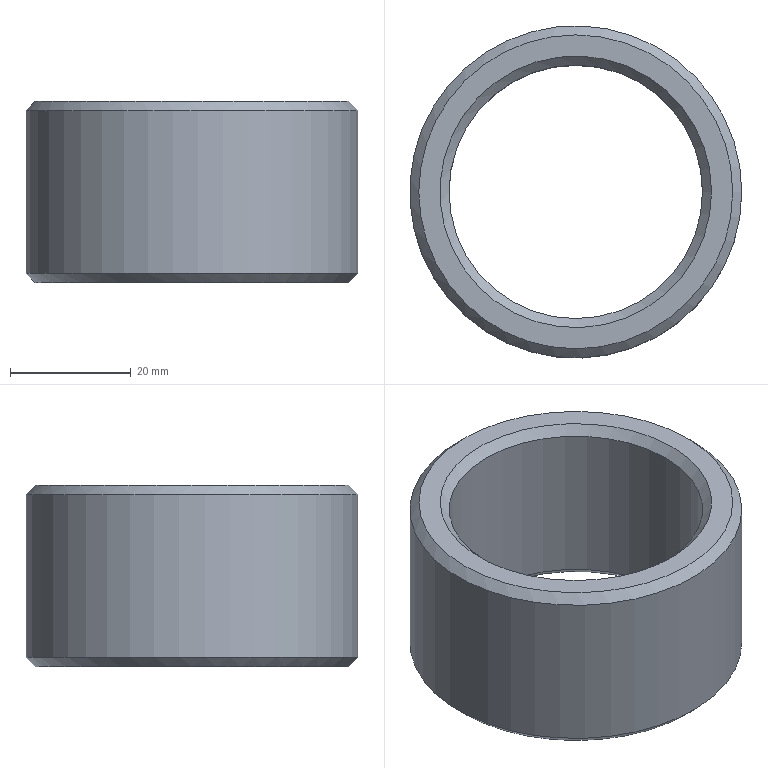Component | NX | BUSHING | 1 solid | 8 faces | box 55 x 55 x 30 mm | volume 29026 mm3 | cone 4 | cylinder 2 | plane 2 | commonest cylinder face diameters 55 x1 42 x1
STEP:
#1=CARTESIAN_POINT('',(0.,0.,0.));
#2=DIRECTION('',(0.,0.,1.));
#3=DIRECTION('',(1.,0.,0.));
#4=AXIS2_PLACEMENT_3D('',#1,#2,#3);
#5=CARTESIAN_POINT('',(61.5,144.033,51.5));
#6=VERTEX_POINT('',#5);
#7=CARTESIAN_POINT('',(34.,144.033,51.5));
#8=DIRECTION('',(0.,0.,1.));
#9=DIRECTION('',(1.,0.,0.));
#10=AXIS2_PLACEMENT_3D('',#7,#8,#9);
#11=CIRCLE('',#10,27.5);
#12=CARTESIAN_POINT('',(34.,144.033,80.));
#13=DIRECTION('',(0.,0.,-1.));
#14=DIRECTION('',(-1.,0.,0.));
#15=AXIS2_PLACEMENT_3D('',#12,#13,#14);
#16=CYLINDRICAL_SURFACE('',#15,27.5);
#17=CARTESIAN_POINT('',(9.425,28.5));
#18=DIRECTION('',(-1.,0.));
#19=VECTOR('',#18,1.);
#20=LINE('',#17,#19);
#21=(GEOMETRIC_REPRESENTATION_CONTEXT(2)PARAMETRIC_REPRESENTATION_CONTEXT()REPRESENTATION_CONTEXT('',''));
#22=DEFINITIONAL_REPRESENTATION('',(#20),#21);
#23=PCURVE('',#16,#22);
#24=CARTESIAN_POINT('',(34.,144.033,51.5));
#25=DIRECTION('',(0.,0.,1.));
#26=DIRECTION('',(1.,0.,0.));
#27=AXIS2_PLACEMENT_3D('',#24,#25,#26);
#28=CONICAL_SURFACE('',#27,27.5,0.7854);
#29=CARTESIAN_POINT('',(0.,0.));
#30=DIRECTION('',(1.,0.));
#31=VECTOR('',#30,1.);
#32=LINE('',#29,#31);
#33=(GEOMETRIC_REPRESENTATION_CONTEXT(2)PARAMETRIC_REPRESENTATION_CONTEXT()REPRESENTATION_CONTEXT('',''));
#34=DEFINITIONAL_REPRESENTATION('',(#32),#33);
#35=PCURVE('',#28,#34);
#36=SURFACE_CURVE('',#11,(#23,#35),.PCURVE_S1.);
#37=EDGE_CURVE('',#6,#6,#36,.T.);
#38=ORIENTED_EDGE('',*,*,#37,.T.);
#39=CARTESIAN_POINT('',(61.5,144.033,78.5));
#40=VERTEX_POINT('',#39);
#41=CARTESIAN_POINT('',(61.5,144.033,78.5));
#42=CARTESIAN_POINT('',(61.5,144.033,51.5));
#43=B_SPLINE_CURVE_WITH_KNOTS('',1,(#41,#42),.UNSPECIFIED.,.F.,.F.,(2,2),(1.5,28.5),.PIECEWISE_BEZIER_KNOTS.);
#44=CARTESIAN_POINT('',(3.142,0.));
#45=DIRECTION('',(0.,1.));
#46=VECTOR('',#45,1.);
#47=LINE('',#44,#46);
#48=(GEOMETRIC_REPRESENTATION_CONTEXT(2)PARAMETRIC_REPRESENTATION_CONTEXT()REPRESENTATION_CONTEXT('',''));
#49=DEFINITIONAL_REPRESENTATION('',(#47),#48);
#50=PCURVE('',#16,#49);
#51=CARTESIAN_POINT('',(9.425,0.));
#52=DIRECTION('',(0.,1.));
#53=VECTOR('',#52,1.);
#54=LINE('',#51,#53);
#55=(GEOMETRIC_REPRESENTATION_CONTEXT(2)PARAMETRIC_REPRESENTATION_CONTEXT()REPRESENTATION_CONTEXT('',''));
#56=DEFINITIONAL_REPRESENTATION('',(#54),#55);
#57=PCURVE('',#16,#56);
#58=SEAM_CURVE('',#43,(#50,#57),.PCURVE_S1.);
#59=EDGE_CURVE('',#40,#6,#58,.T.);
#60=ORIENTED_EDGE('',*,*,#59,.F.);
#61=CARTESIAN_POINT('',(34.,144.033,78.5));
#62=DIRECTION('',(0.,0.,-1.));
#63=DIRECTION('',(1.,0.,0.));
#64=AXIS2_PLACEMENT_3D('',#61,#62,#63);
#65=CIRCLE('',#64,27.5);
#66=CARTESIAN_POINT('',(3.142,1.5));
#67=DIRECTION('',(1.,0.));
#68=VECTOR('',#67,1.);
#69=LINE('',#66,#68);
#70=(GEOMETRIC_REPRESENTATION_CONTEXT(2)PARAMETRIC_REPRESENTATION_CONTEXT()REPRESENTATION_CONTEXT('',''));
#71=DEFINITIONAL_REPRESENTATION('',(#69),#70);
#72=PCURVE('',#16,#71);
#73=CARTESIAN_POINT('',(34.,144.033,80.));
#74=DIRECTION('',(0.,0.,-1.));
#75=DIRECTION('',(-1.,0.,0.));
#76=AXIS2_PLACEMENT_3D('',#73,#74,#75);
#77=CONICAL_SURFACE('',#76,26.,0.7854);
#78=CARTESIAN_POINT('',(3.142,1.5));
#79=DIRECTION('',(1.,0.));
#80=VECTOR('',#79,1.);
#81=LINE('',#78,#80);
#82=(GEOMETRIC_REPRESENTATION_CONTEXT(2)PARAMETRIC_REPRESENTATION_CONTEXT()REPRESENTATION_CONTEXT('',''));
#83=DEFINITIONAL_REPRESENTATION('',(#81),#82);
#84=PCURVE('',#77,#83);
#85=SURFACE_CURVE('',#65,(#72,#84),.PCURVE_S1.);
#86=EDGE_CURVE('',#40,#40,#85,.T.);
#87=ORIENTED_EDGE('',*,*,#86,.T.);
#88=ORIENTED_EDGE('',*,*,#59,.T.);
#89=EDGE_LOOP('',(#38,#60,#87,#88));
#90=FACE_BOUND('',#89,.T.);
#91=ADVANCED_FACE('',(#90),#16,.T.);
#92=CARTESIAN_POINT('',(55.,144.033,51.5));
#93=VERTEX_POINT('',#92);
#94=CARTESIAN_POINT('',(34.,144.033,51.5));
#95=DIRECTION('',(0.,0.,-1.));
#96=DIRECTION('',(1.,0.,0.));
#97=AXIS2_PLACEMENT_3D('',#94,#95,#96);
#98=CIRCLE('',#97,21.);
#99=CARTESIAN_POINT('',(34.,144.033,80.));
#100=DIRECTION('',(0.,0.,-1.));
#101=DIRECTION('',(-1.,0.,0.));
#102=AXIS2_PLACEMENT_3D('',#99,#100,#101);
#103=CYLINDRICAL_SURFACE('',#102,21.);
#104=CARTESIAN_POINT('',(3.142,28.5));
#105=DIRECTION('',(1.,0.));
#106=VECTOR('',#105,1.);
#107=LINE('',#104,#106);
#108=(GEOMETRIC_REPRESENTATION_CONTEXT(2)PARAMETRIC_REPRESENTATION_CONTEXT()REPRESENTATION_CONTEXT('',''));
#109=DEFINITIONAL_REPRESENTATION('',(#107),#108);
#110=PCURVE('',#103,#109);
#111=CARTESIAN_POINT('',(34.,144.033,50.));
#112=DIRECTION('',(0.,0.,-1.));
#113=DIRECTION('',(-1.,0.,0.));
#114=AXIS2_PLACEMENT_3D('',#111,#112,#113);
#115=CONICAL_SURFACE('',#114,22.5,0.7854);
#116=CARTESIAN_POINT('',(3.142,-1.5));
#117=DIRECTION('',(1.,0.));
#118=VECTOR('',#117,1.);
#119=LINE('',#116,#118);
#120=(GEOMETRIC_REPRESENTATION_CONTEXT(2)PARAMETRIC_REPRESENTATION_CONTEXT()REPRESENTATION_CONTEXT('',''));
#121=DEFINITIONAL_REPRESENTATION('',(#119),#120);
#122=PCURVE('',#115,#121);
#123=SURFACE_CURVE('',#98,(#110,#122),.PCURVE_S1.);
#124=EDGE_CURVE('',#93,#93,#123,.T.);
#125=ORIENTED_EDGE('',*,*,#124,.F.);
#126=CARTESIAN_POINT('',(55.,144.033,78.5));
#127=VERTEX_POINT('',#126);
#128=CARTESIAN_POINT('',(55.,144.033,78.5));
#129=CARTESIAN_POINT('',(55.,144.033,51.5));
#130=B_SPLINE_CURVE_WITH_KNOTS('',1,(#128,#129),.UNSPECIFIED.,.F.,.F.,(2,2),(1.5,28.5),.PIECEWISE_BEZIER_KNOTS.);
#131=CARTESIAN_POINT('',(3.142,0.));
#132=DIRECTION('',(0.,1.));
#133=VECTOR('',#132,1.);
#134=LINE('',#131,#133);
#135=(GEOMETRIC_REPRESENTATION_CONTEXT(2)PARAMETRIC_REPRESENTATION_CONTEXT()REPRESENTATION_CONTEXT('',''));
#136=DEFINITIONAL_REPRESENTATION('',(#134),#135);
#137=PCURVE('',#103,#136);
#138=CARTESIAN_POINT('',(9.425,0.));
#139=DIRECTION('',(0.,1.));
#140=VECTOR('',#139,1.);
#141=LINE('',#138,#140);
#142=(GEOMETRIC_REPRESENTATION_CONTEXT(2)PARAMETRIC_REPRESENTATION_CONTEXT()REPRESENTATION_CONTEXT('',''));
#143=DEFINITIONAL_REPRESENTATION('',(#141),#142);
#144=PCURVE('',#103,#143);
#145=SEAM_CURVE('',#130,(#137,#144),.PCURVE_S1.);
#146=EDGE_CURVE('',#127,#93,#145,.T.);
#147=ORIENTED_EDGE('',*,*,#146,.F.);
#148=CARTESIAN_POINT('',(34.,144.033,78.5));
#149=DIRECTION('',(0.,0.,1.));
#150=DIRECTION('',(1.,0.,0.));
#151=AXIS2_PLACEMENT_3D('',#148,#149,#150);
#152=CIRCLE('',#151,21.);
#153=CARTESIAN_POINT('',(9.425,1.5));
#154=DIRECTION('',(-1.,0.));
#155=VECTOR('',#154,1.);
#156=LINE('',#153,#155);
#157=(GEOMETRIC_REPRESENTATION_CONTEXT(2)PARAMETRIC_REPRESENTATION_CONTEXT()REPRESENTATION_CONTEXT('',''));
#158=DEFINITIONAL_REPRESENTATION('',(#156),#157);
#159=PCURVE('',#103,#158);
#160=CARTESIAN_POINT('',(34.,144.033,78.5));
#161=DIRECTION('',(0.,0.,1.));
#162=DIRECTION('',(1.,0.,0.));
#163=AXIS2_PLACEMENT_3D('',#160,#161,#162);
#164=CONICAL_SURFACE('',#163,21.,0.7854);
#165=CARTESIAN_POINT('',(0.,0.));
#166=DIRECTION('',(1.,0.));
#167=VECTOR('',#166,1.);
#168=LINE('',#165,#167);
#169=(GEOMETRIC_REPRESENTATION_CONTEXT(2)PARAMETRIC_REPRESENTATION_CONTEXT()REPRESENTATION_CONTEXT('',''));
#170=DEFINITIONAL_REPRESENTATION('',(#168),#169);
#171=PCURVE('',#164,#170);
#172=SURFACE_CURVE('',#152,(#159,#171),.PCURVE_S1.);
#173=EDGE_CURVE('',#127,#127,#172,.T.);
#174=ORIENTED_EDGE('',*,*,#173,.F.);
#175=ORIENTED_EDGE('',*,*,#146,.T.);
#176=EDGE_LOOP('',(#125,#147,#174,#175));
#177=FACE_BOUND('',#176,.F.);
#178=ADVANCED_FACE('',(#177),#103,.F.);
#179=CARTESIAN_POINT('',(56.5,144.033,80.));
#180=VERTEX_POINT('',#179);
#181=CARTESIAN_POINT('',(34.,144.033,80.));
#182=DIRECTION('',(0.,0.,-1.));
#183=DIRECTION('',(1.,0.,0.));
#184=AXIS2_PLACEMENT_3D('',#181,#182,#183);
#185=CIRCLE('',#184,22.5);
#186=CARTESIAN_POINT('',(34.,144.033,80.));
#187=DIRECTION('',(0.,0.,1.));
#188=DIRECTION('',(1.,0.,0.));
#189=AXIS2_PLACEMENT_3D('',#186,#187,#188);
#190=PLANE('',#189);
#191=CARTESIAN_POINT('',(22.5,0.));
#192=CARTESIAN_POINT('',(22.5,-38.971));
#193=CARTESIAN_POINT('',(-11.25,-19.486));
#194=CARTESIAN_POINT('',(-45.,-0.));
#195=CARTESIAN_POINT('',(-11.25,19.486));
#196=CARTESIAN_POINT('',(22.5,38.971));
#197=CARTESIAN_POINT('',(22.5,0.));
#198=(BOUNDED_CURVE()B_SPLINE_CURVE(2,(#191,#192,#193,#194,#195,#196,#197),.UNSPECIFIED.,.T.,.F.)B_SPLINE_CURVE_WITH_KNOTS((1,2,2,2,2,1),(-2.094,0.,2.094,4.189,6.283,8.378),.UNSPECIFIED.)CURVE()GEOMETRIC_REPRESENTATION_ITEM()RATIONAL_B_SPLINE_CURVE((1.,0.5,1.,0.5,1.,0.5,1.))REPRESENTATION_ITEM(''));
#199=(GEOMETRIC_REPRESENTATION_CONTEXT(2)PARAMETRIC_REPRESENTATION_CONTEXT()REPRESENTATION_CONTEXT('',''));
#200=DEFINITIONAL_REPRESENTATION('',(#198),#199);
#201=PCURVE('',#190,#200);
#202=CARTESIAN_POINT('',(6.283,1.5));
#203=DIRECTION('',(-1.,0.));
#204=VECTOR('',#203,1.);
#205=LINE('',#202,#204);
#206=(GEOMETRIC_REPRESENTATION_CONTEXT(2)PARAMETRIC_REPRESENTATION_CONTEXT()REPRESENTATION_CONTEXT('',''));
#207=DEFINITIONAL_REPRESENTATION('',(#205),#206);
#208=PCURVE('',#164,#207);
#209=SURFACE_CURVE('',#185,(#201,#208),.PCURVE_S1.);
#210=EDGE_CURVE('',#180,#180,#209,.T.);
#211=ORIENTED_EDGE('',*,*,#210,.T.);
#212=EDGE_LOOP('',(#211));
#213=FACE_BOUND('',#212,.T.);
#214=CARTESIAN_POINT('',(60.,144.033,80.));
#215=VERTEX_POINT('',#214);
#216=CARTESIAN_POINT('',(34.,144.033,80.));
#217=DIRECTION('',(0.,0.,1.));
#218=DIRECTION('',(1.,0.,0.));
#219=AXIS2_PLACEMENT_3D('',#216,#217,#218);
#220=CIRCLE('',#219,26.);
#221=CARTESIAN_POINT('',(0.,0.));
#222=DIRECTION('',(1.,0.));
#223=AXIS2_PLACEMENT_2D('',#221,#222);
#224=CIRCLE('',#223,26.);
#225=(GEOMETRIC_REPRESENTATION_CONTEXT(2)PARAMETRIC_REPRESENTATION_CONTEXT()REPRESENTATION_CONTEXT('',''));
#226=DEFINITIONAL_REPRESENTATION('',(#224),#225);
#227=PCURVE('',#190,#226);
#228=CARTESIAN_POINT('',(9.425,0.));
#229=DIRECTION('',(-1.,0.));
#230=VECTOR('',#229,1.);
#231=LINE('',#228,#230);
#232=(GEOMETRIC_REPRESENTATION_CONTEXT(2)PARAMETRIC_REPRESENTATION_CONTEXT()REPRESENTATION_CONTEXT('',''));
#233=DEFINITIONAL_REPRESENTATION('',(#231),#232);
#234=PCURVE('',#77,#233);
#235=SURFACE_CURVE('',#220,(#227,#234),.PCURVE_S1.);
#236=EDGE_CURVE('',#215,#215,#235,.T.);
#237=ORIENTED_EDGE('',*,*,#236,.T.);
#238=EDGE_LOOP('',(#237));
#239=FACE_BOUND('',#238,.T.);
#240=ADVANCED_FACE('',(#213,#239),#190,.T.);
#241=CARTESIAN_POINT('',(56.5,144.033,50.));
#242=VERTEX_POINT('',#241);
#243=CARTESIAN_POINT('',(34.,144.033,50.));
#244=DIRECTION('',(0.,0.,1.));
#245=DIRECTION('',(1.,0.,0.));
#246=AXIS2_PLACEMENT_3D('',#243,#244,#245);
#247=CIRCLE('',#246,22.5);
#248=CARTESIAN_POINT('',(34.,144.033,50.));
#249=DIRECTION('',(0.,0.,1.));
#250=DIRECTION('',(1.,0.,0.));
#251=AXIS2_PLACEMENT_3D('',#248,#249,#250);
#252=PLANE('',#251);
#253=CARTESIAN_POINT('',(0.,0.));
#254=DIRECTION('',(1.,0.));
#255=AXIS2_PLACEMENT_2D('',#253,#254);
#256=CIRCLE('',#255,22.5);
#257=(GEOMETRIC_REPRESENTATION_CONTEXT(2)PARAMETRIC_REPRESENTATION_CONTEXT()REPRESENTATION_CONTEXT('',''));
#258=DEFINITIONAL_REPRESENTATION('',(#256),#257);
#259=PCURVE('',#252,#258);
#260=CARTESIAN_POINT('',(9.425,0.));
#261=DIRECTION('',(-1.,0.));
#262=VECTOR('',#261,1.);
#263=LINE('',#260,#262);
#264=(GEOMETRIC_REPRESENTATION_CONTEXT(2)PARAMETRIC_REPRESENTATION_CONTEXT()REPRESENTATION_CONTEXT('',''));
#265=DEFINITIONAL_REPRESENTATION('',(#263),#264);
#266=PCURVE('',#115,#265);
#267=SURFACE_CURVE('',#247,(#259,#266),.PCURVE_S1.);
#268=EDGE_CURVE('',#242,#242,#267,.T.);
#269=ORIENTED_EDGE('',*,*,#268,.T.);
#270=EDGE_LOOP('',(#269));
#271=FACE_BOUND('',#270,.T.);
#272=CARTESIAN_POINT('',(60.,144.033,50.));
#273=VERTEX_POINT('',#272);
#274=CARTESIAN_POINT('',(34.,144.033,50.));
#275=DIRECTION('',(0.,0.,-1.));
#276=DIRECTION('',(1.,0.,0.));
#277=AXIS2_PLACEMENT_3D('',#274,#275,#276);
#278=CIRCLE('',#277,26.);
#279=CARTESIAN_POINT('',(26.,0.));
#280=CARTESIAN_POINT('',(26.,-45.033));
#281=CARTESIAN_POINT('',(-13.,-22.517));
#282=CARTESIAN_POINT('',(-52.,-0.));
#283=CARTESIAN_POINT('',(-13.,22.517));
#284=CARTESIAN_POINT('',(26.,45.033));
#285=CARTESIAN_POINT('',(26.,0.));
#286=(BOUNDED_CURVE()B_SPLINE_CURVE(2,(#279,#280,#281,#282,#283,#284,#285),.UNSPECIFIED.,.T.,.F.)B_SPLINE_CURVE_WITH_KNOTS((1,2,2,2,2,1),(-2.094,0.,2.094,4.189,6.283,8.378),.UNSPECIFIED.)CURVE()GEOMETRIC_REPRESENTATION_ITEM()RATIONAL_B_SPLINE_CURVE((1.,0.5,1.,0.5,1.,0.5,1.))REPRESENTATION_ITEM(''));
#287=(GEOMETRIC_REPRESENTATION_CONTEXT(2)PARAMETRIC_REPRESENTATION_CONTEXT()REPRESENTATION_CONTEXT('',''));
#288=DEFINITIONAL_REPRESENTATION('',(#286),#287);
#289=PCURVE('',#252,#288);
#290=CARTESIAN_POINT('',(6.283,-1.5));
#291=DIRECTION('',(-1.,0.));
#292=VECTOR('',#291,1.);
#293=LINE('',#290,#292);
#294=(GEOMETRIC_REPRESENTATION_CONTEXT(2)PARAMETRIC_REPRESENTATION_CONTEXT()REPRESENTATION_CONTEXT('',''));
#295=DEFINITIONAL_REPRESENTATION('',(#293),#294);
#296=PCURVE('',#28,#295);
#297=SURFACE_CURVE('',#278,(#289,#296),.PCURVE_S1.);
#298=EDGE_CURVE('',#273,#273,#297,.T.);
#299=ORIENTED_EDGE('',*,*,#298,.T.);
#300=EDGE_LOOP('',(#299));
#301=FACE_BOUND('',#300,.T.);
#302=ADVANCED_FACE('',(#271,#301),#252,.F.);
#303=ORIENTED_EDGE('',*,*,#124,.T.);
#304=CARTESIAN_POINT('',(55.,144.033,51.5));
#305=CARTESIAN_POINT('',(56.5,144.033,50.));
#306=B_SPLINE_CURVE_WITH_KNOTS('',1,(#304,#305),.UNSPECIFIED.,.F.,.F.,(2,2),(-2.121,0.),.PIECEWISE_BEZIER_KNOTS.);
#307=CARTESIAN_POINT('',(9.425,0.));
#308=DIRECTION('',(0.,1.));
#309=VECTOR('',#308,1.);
#310=LINE('',#307,#309);
#311=(GEOMETRIC_REPRESENTATION_CONTEXT(2)PARAMETRIC_REPRESENTATION_CONTEXT()REPRESENTATION_CONTEXT('',''));
#312=DEFINITIONAL_REPRESENTATION('',(#310),#311);
#313=PCURVE('',#115,#312);
#314=CARTESIAN_POINT('',(3.142,0.));
#315=DIRECTION('',(0.,1.));
#316=VECTOR('',#315,1.);
#317=LINE('',#314,#316);
#318=(GEOMETRIC_REPRESENTATION_CONTEXT(2)PARAMETRIC_REPRESENTATION_CONTEXT()REPRESENTATION_CONTEXT('',''));
#319=DEFINITIONAL_REPRESENTATION('',(#317),#318);
#320=PCURVE('',#115,#319);
#321=SEAM_CURVE('',#306,(#313,#320),.PCURVE_S1.);
#322=EDGE_CURVE('',#93,#242,#321,.T.);
#323=ORIENTED_EDGE('',*,*,#322,.T.);
#324=ORIENTED_EDGE('',*,*,#268,.T.);
#325=ORIENTED_EDGE('',*,*,#322,.F.);
#326=EDGE_LOOP('',(#303,#323,#324,#325));
#327=FACE_BOUND('',#326,.F.);
#328=ADVANCED_FACE('',(#327),#115,.F.);
#329=ORIENTED_EDGE('',*,*,#298,.F.);
#330=CARTESIAN_POINT('',(60.,144.033,50.));
#331=CARTESIAN_POINT('',(61.5,144.033,51.5));
#332=B_SPLINE_CURVE_WITH_KNOTS('',1,(#330,#331),.UNSPECIFIED.,.F.,.F.,(2,2),(-2.121,0.),.PIECEWISE_BEZIER_KNOTS.);
#333=CARTESIAN_POINT('',(6.283,0.));
#334=DIRECTION('',(0.,1.));
#335=VECTOR('',#334,1.);
#336=LINE('',#333,#335);
#337=(GEOMETRIC_REPRESENTATION_CONTEXT(2)PARAMETRIC_REPRESENTATION_CONTEXT()REPRESENTATION_CONTEXT('',''));
#338=DEFINITIONAL_REPRESENTATION('',(#336),#337);
#339=PCURVE('',#28,#338);
#340=CARTESIAN_POINT('',(0.,0.));
#341=DIRECTION('',(0.,1.));
#342=VECTOR('',#341,1.);
#343=LINE('',#340,#342);
#344=(GEOMETRIC_REPRESENTATION_CONTEXT(2)PARAMETRIC_REPRESENTATION_CONTEXT()REPRESENTATION_CONTEXT('',''));
#345=DEFINITIONAL_REPRESENTATION('',(#343),#344);
#346=PCURVE('',#28,#345);
#347=SEAM_CURVE('',#332,(#339,#346),.PCURVE_S1.);
#348=EDGE_CURVE('',#273,#6,#347,.T.);
#349=ORIENTED_EDGE('',*,*,#348,.T.);
#350=ORIENTED_EDGE('',*,*,#37,.F.);
#351=ORIENTED_EDGE('',*,*,#348,.F.);
#352=EDGE_LOOP('',(#329,#349,#350,#351));
#353=FACE_BOUND('',#352,.T.);
#354=ADVANCED_FACE('',(#353),#28,.T.);
#355=ORIENTED_EDGE('',*,*,#210,.T.);
#356=CARTESIAN_POINT('',(55.,144.033,78.5));
#357=CARTESIAN_POINT('',(56.5,144.033,80.));
#358=B_SPLINE_CURVE_WITH_KNOTS('',1,(#356,#357),.UNSPECIFIED.,.F.,.F.,(2,2),(0.,2.121),.PIECEWISE_BEZIER_KNOTS.);
#359=CARTESIAN_POINT('',(0.,0.));
#360=DIRECTION('',(0.,1.));
#361=VECTOR('',#360,1.);
#362=LINE('',#359,#361);
#363=(GEOMETRIC_REPRESENTATION_CONTEXT(2)PARAMETRIC_REPRESENTATION_CONTEXT()REPRESENTATION_CONTEXT('',''));
#364=DEFINITIONAL_REPRESENTATION('',(#362),#363);
#365=PCURVE('',#164,#364);
#366=CARTESIAN_POINT('',(6.283,0.));
#367=DIRECTION('',(0.,1.));
#368=VECTOR('',#367,1.);
#369=LINE('',#366,#368);
#370=(GEOMETRIC_REPRESENTATION_CONTEXT(2)PARAMETRIC_REPRESENTATION_CONTEXT()REPRESENTATION_CONTEXT('',''));
#371=DEFINITIONAL_REPRESENTATION('',(#369),#370);
#372=PCURVE('',#164,#371);
#373=SEAM_CURVE('',#358,(#365,#372),.PCURVE_S1.);
#374=EDGE_CURVE('',#127,#180,#373,.T.);
#375=ORIENTED_EDGE('',*,*,#374,.F.);
#376=ORIENTED_EDGE('',*,*,#173,.T.);
#377=ORIENTED_EDGE('',*,*,#374,.T.);
#378=EDGE_LOOP('',(#355,#375,#376,#377));
#379=FACE_BOUND('',#378,.F.);
#380=ADVANCED_FACE('',(#379),#164,.F.);
#381=ORIENTED_EDGE('',*,*,#86,.F.);
#382=CARTESIAN_POINT('',(60.,144.033,80.));
#383=CARTESIAN_POINT('',(61.5,144.033,78.5));
#384=B_SPLINE_CURVE_WITH_KNOTS('',1,(#382,#383),.UNSPECIFIED.,.F.,.F.,(2,2),(0.,2.121),.PIECEWISE_BEZIER_KNOTS.);
#385=CARTESIAN_POINT('',(3.142,0.));
#386=DIRECTION('',(0.,1.));
#387=VECTOR('',#386,1.);
#388=LINE('',#385,#387);
#389=(GEOMETRIC_REPRESENTATION_CONTEXT(2)PARAMETRIC_REPRESENTATION_CONTEXT()REPRESENTATION_CONTEXT('',''));
#390=DEFINITIONAL_REPRESENTATION('',(#388),#389);
#391=PCURVE('',#77,#390);
#392=CARTESIAN_POINT('',(9.425,0.));
#393=DIRECTION('',(0.,1.));
#394=VECTOR('',#393,1.);
#395=LINE('',#392,#394);
#396=(GEOMETRIC_REPRESENTATION_CONTEXT(2)PARAMETRIC_REPRESENTATION_CONTEXT()REPRESENTATION_CONTEXT('',''));
#397=DEFINITIONAL_REPRESENTATION('',(#395),#396);
#398=PCURVE('',#77,#397);
#399=SEAM_CURVE('',#384,(#391,#398),.PCURVE_S1.);
#400=EDGE_CURVE('',#215,#40,#399,.T.);
#401=ORIENTED_EDGE('',*,*,#400,.F.);
#402=ORIENTED_EDGE('',*,*,#236,.F.);
#403=ORIENTED_EDGE('',*,*,#400,.T.);
#404=EDGE_LOOP('',(#381,#401,#402,#403));
#405=FACE_BOUND('',#404,.T.);
#406=ADVANCED_FACE('',(#405),#77,.T.);
#407=CLOSED_SHELL('',(#91,#178,#240,#302,#328,#354,#380,#406));
#408=MANIFOLD_SOLID_BREP('',#407);
#409=(LENGTH_UNIT()NAMED_UNIT(*)SI_UNIT(.MILLI.,.METRE.));
#410=UNCERTAINTY_MEASURE_WITH_UNIT(LENGTH_MEASURE(0.00001),#409,'','');
#411=(NAMED_UNIT(*)PLANE_ANGLE_UNIT()SI_UNIT($,.RADIAN.));
#412=(NAMED_UNIT(*)SI_UNIT($,.STERADIAN.)SOLID_ANGLE_UNIT());
#413=(GEOMETRIC_REPRESENTATION_CONTEXT(3)GLOBAL_UNCERTAINTY_ASSIGNED_CONTEXT((#410))GLOBAL_UNIT_ASSIGNED_CONTEXT((#409,#411,#412))REPRESENTATION_CONTEXT('',''));
#414=ADVANCED_BREP_SHAPE_REPRESENTATION('',(#4,#408),#413);